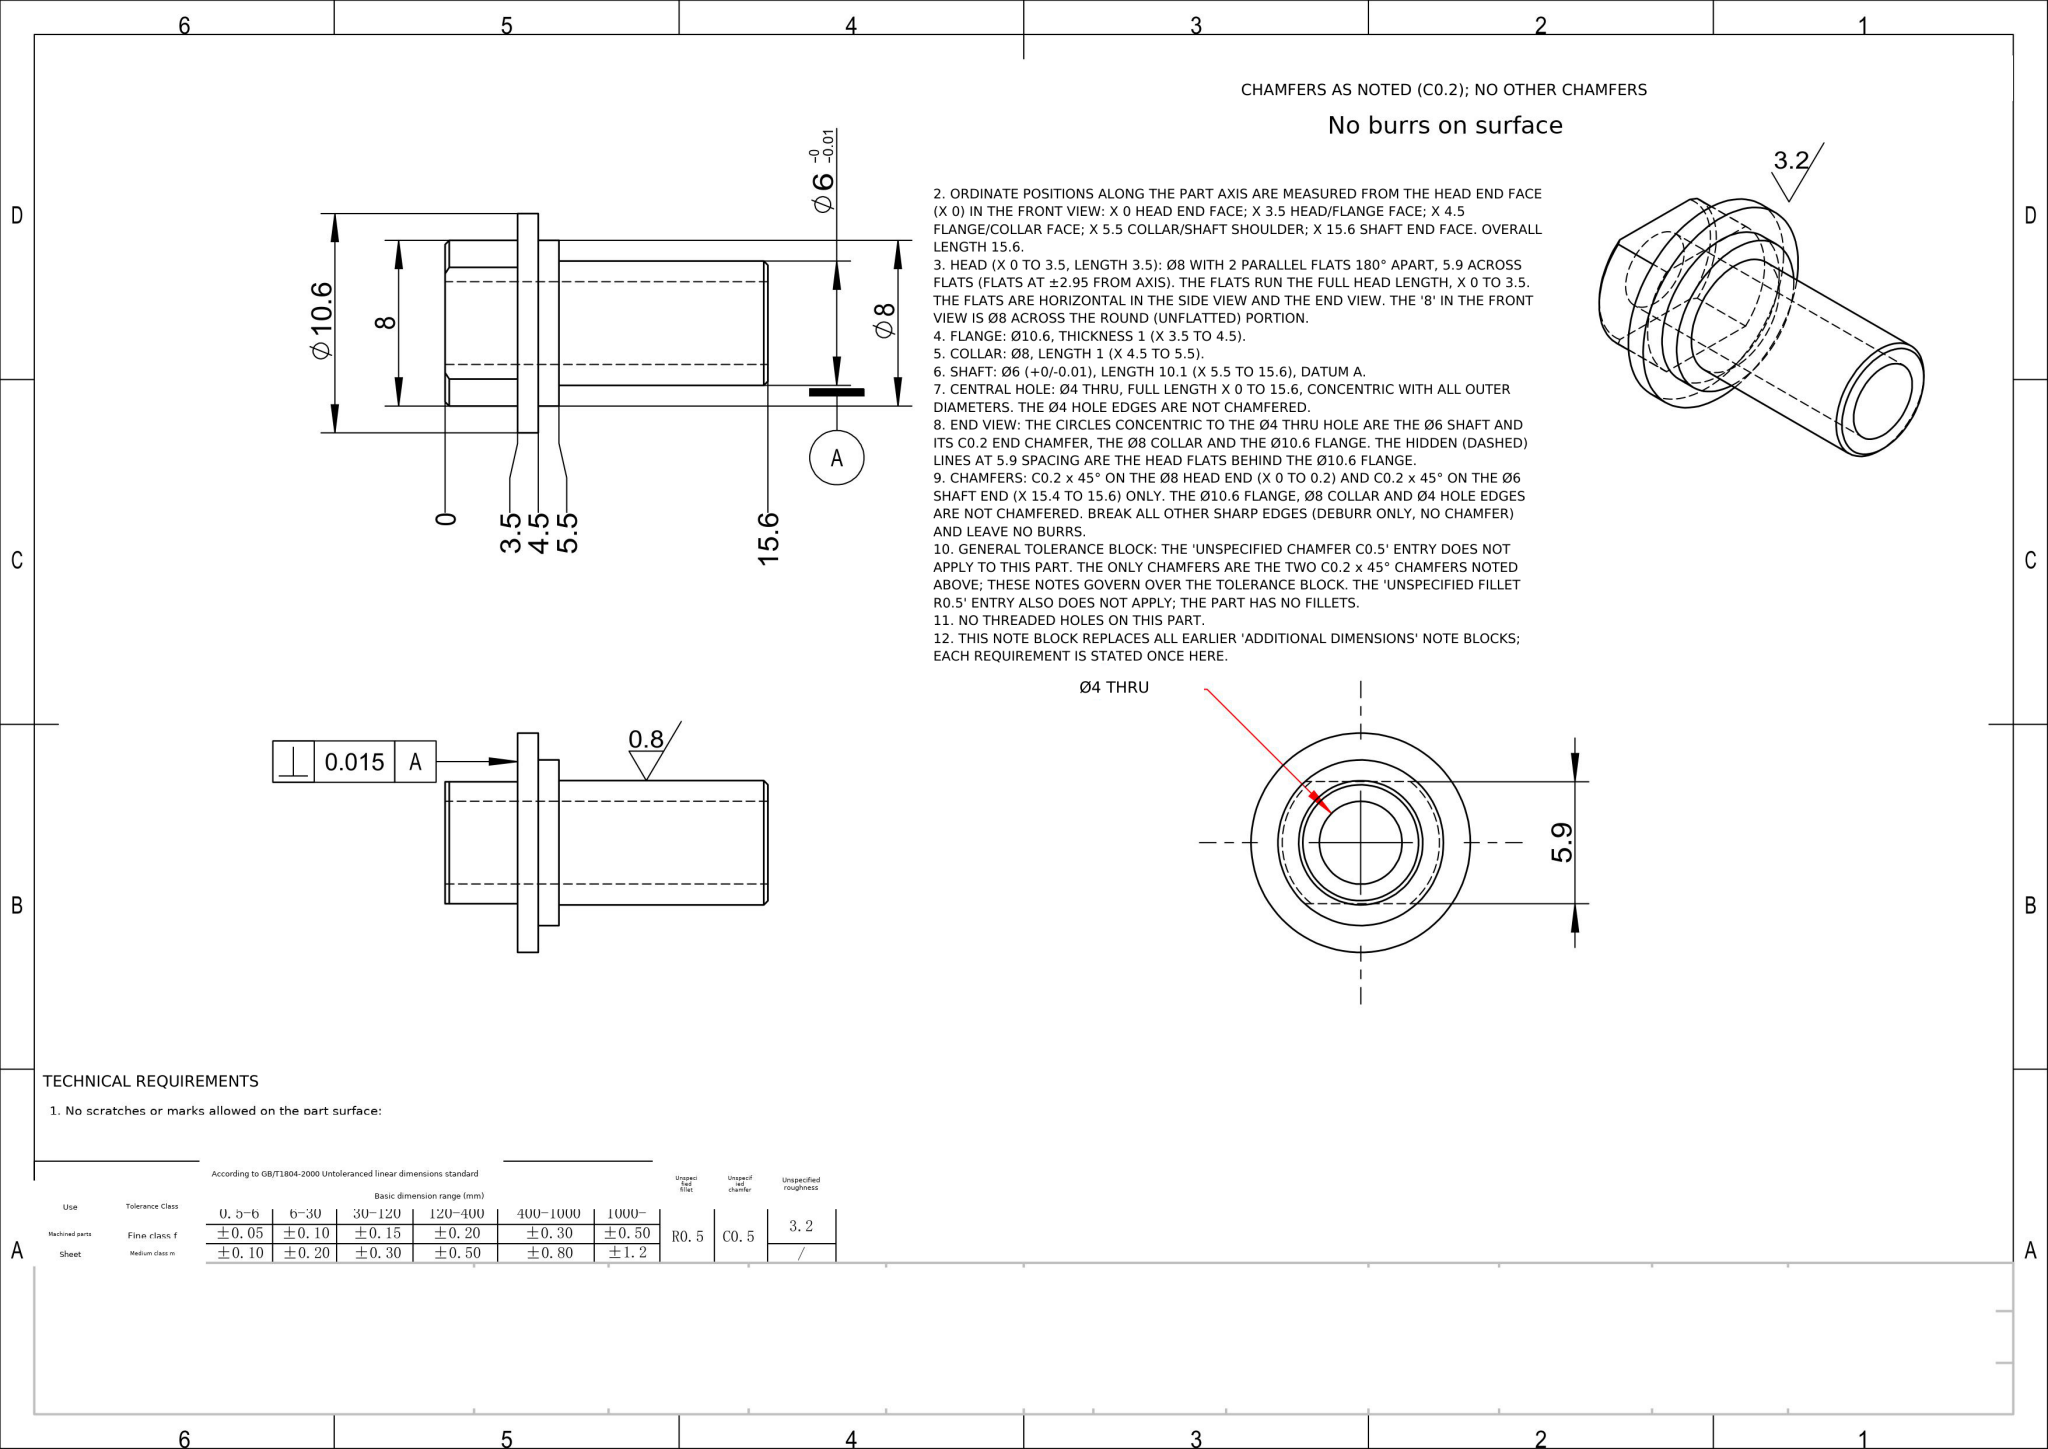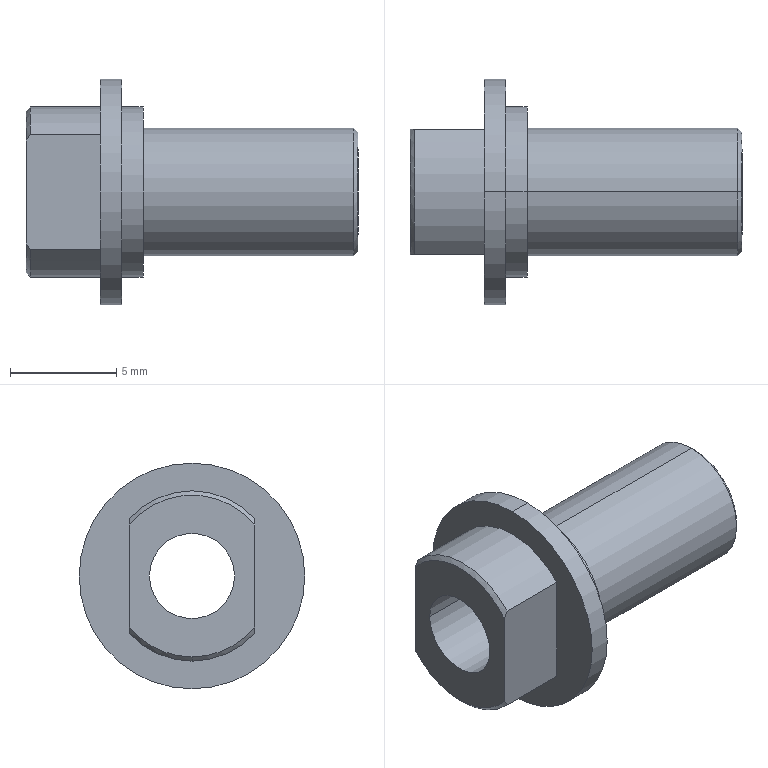Part | NX | mm | 1 solid | 23 faces | box 15.6 x 10.6 x 10.6 mm | volume 376 mm3 | cylinder 11 | plane 7 | cone 5 | commonest cylinder face diameters 8 x5 4 x2 6 x2 10.6 x2
STEP:
#1=COLOUR_RGB('',0.7529,0.7529,0.7529);
#2=FILL_AREA_STYLE_COLOUR('',#1);
#3=FILL_AREA_STYLE('',(#2));
#4=SURFACE_STYLE_FILL_AREA(#3);
#5=SURFACE_SIDE_STYLE('',(#4));
#6=SURFACE_STYLE_USAGE(.BOTH.,#5);
#7=PRESENTATION_STYLE_ASSIGNMENT((#6));
#8=CARTESIAN_POINT('',(-0.,-2.,0.));
#9=VERTEX_POINT('',#8);
#10=CARTESIAN_POINT('',(-0.,2.,0.));
#11=VERTEX_POINT('',#10);
#12=CARTESIAN_POINT('',(-0.,0.,0.));
#13=DIRECTION('',(1.,-0.,0.));
#14=DIRECTION('',(0.,1.,0.));
#15=AXIS2_PLACEMENT_3D('',#12,#13,#14);
#16=CIRCLE('',#15,2.);
#17=EDGE_CURVE('',#9,#11,#16,.T.);
#18=ORIENTED_EDGE('',*,*,#17,.F.);
#19=CARTESIAN_POINT('',(15.6,-2.,0.));
#20=VERTEX_POINT('',#19);
#21=CARTESIAN_POINT('',(-6.035,-2.,0.));
#22=DIRECTION('',(1.,-0.,0.));
#23=VECTOR('',#22,1000.);
#24=LINE('',#21,#23);
#25=EDGE_CURVE('',#9,#20,#24,.T.);
#26=ORIENTED_EDGE('',*,*,#25,.T.);
#27=CARTESIAN_POINT('',(15.6,2.,0.));
#28=VERTEX_POINT('',#27);
#29=CARTESIAN_POINT('',(15.6,-0.,0.));
#30=DIRECTION('',(-1.,0.,0.));
#31=DIRECTION('',(0.,1.,0.));
#32=AXIS2_PLACEMENT_3D('',#29,#30,#31);
#33=CIRCLE('',#32,2.);
#34=EDGE_CURVE('',#28,#20,#33,.T.);
#35=ORIENTED_EDGE('',*,*,#34,.F.);
#36=CARTESIAN_POINT('',(-6.035,2.,0.));
#37=DIRECTION('',(1.,-0.,0.));
#38=VECTOR('',#37,1000.);
#39=LINE('',#36,#38);
#40=EDGE_CURVE('',#11,#28,#39,.T.);
#41=ORIENTED_EDGE('',*,*,#40,.F.);
#42=EDGE_LOOP('',(#18,#26,#35,#41));
#43=FACE_OUTER_BOUND('',#42,.T.);
#44=CARTESIAN_POINT('',(-6.035,0.,0.));
#45=DIRECTION('',(1.,-0.,0.));
#46=DIRECTION('',(0.,1.,0.));
#47=AXIS2_PLACEMENT_3D('',#44,#45,#46);
#48=CYLINDRICAL_SURFACE('',#47,2.);
#49=ADVANCED_FACE('',(#43),#48,.F.);
#50=CARTESIAN_POINT('',(0.,0.,-3.8));
#51=VERTEX_POINT('',#50);
#52=CARTESIAN_POINT('',(-0.,-2.95,-2.395));
#53=VERTEX_POINT('',#52);
#54=CARTESIAN_POINT('',(0.,0.,0.));
#55=DIRECTION('',(-1.,0.,0.));
#56=DIRECTION('',(0.,0.,-1.));
#57=AXIS2_PLACEMENT_3D('',#54,#55,#56);
#58=CIRCLE('',#57,3.8);
#59=EDGE_CURVE('',#51,#53,#58,.T.);
#60=ORIENTED_EDGE('',*,*,#59,.F.);
#61=CARTESIAN_POINT('',(0.2,-0.,-4.));
#62=VERTEX_POINT('',#61);
#63=CARTESIAN_POINT('',(0.2,0.,-4.));
#64=DIRECTION('',(0.7071,0.,-0.7071));
#65=VECTOR('',#64,1000.);
#66=LINE('',#63,#65);
#67=EDGE_CURVE('',#51,#62,#66,.T.);
#68=ORIENTED_EDGE('',*,*,#67,.T.);
#69=CARTESIAN_POINT('',(0.2,-2.95,-2.701));
#70=VERTEX_POINT('',#69);
#71=CARTESIAN_POINT('',(0.2,-0.,0.));
#72=DIRECTION('',(-1.,0.,0.));
#73=DIRECTION('',(-0.,1.,0.));
#74=AXIS2_PLACEMENT_3D('',#71,#72,#73);
#75=CIRCLE('',#74,4.);
#76=EDGE_CURVE('',#62,#70,#75,.T.);
#77=ORIENTED_EDGE('',*,*,#76,.T.);
#78=CARTESIAN_POINT('',(0.2,-2.95,-2.701));
#79=CARTESIAN_POINT('',(0.1318,-2.95,-2.6));
#80=CARTESIAN_POINT('',(0.06499,-2.95,-2.498));
#81=CARTESIAN_POINT('',(-0.,-2.95,-2.395));
#82=B_SPLINE_CURVE_WITH_KNOTS('',3,(#78,#79,#80,#81),.UNSPECIFIED.,.F.,.F.,(4,4),(0.,0.0003656),.UNSPECIFIED.);
#83=EDGE_CURVE('',#70,#53,#82,.T.);
#84=ORIENTED_EDGE('',*,*,#83,.T.);
#85=EDGE_LOOP('',(#60,#68,#77,#84));
#86=FACE_OUTER_BOUND('',#85,.T.);
#87=CARTESIAN_POINT('',(0.2,0.,0.));
#88=DIRECTION('',(1.,0.,0.));
#89=DIRECTION('',(0.,0.,-1.));
#90=AXIS2_PLACEMENT_3D('',#87,#88,#89);
#91=CONICAL_SURFACE('',#90,4.,0.7854);
#92=ADVANCED_FACE('',(#86),#91,.T.);
#93=CARTESIAN_POINT('',(15.6,0.,-2.8));
#94=VERTEX_POINT('',#93);
#95=CARTESIAN_POINT('',(15.6,0.,2.8));
#96=VERTEX_POINT('',#95);
#97=CARTESIAN_POINT('',(15.6,0.,0.));
#98=DIRECTION('',(1.,0.,0.));
#99=DIRECTION('',(0.,0.,1.));
#100=AXIS2_PLACEMENT_3D('',#97,#98,#99);
#101=CIRCLE('',#100,2.8);
#102=EDGE_CURVE('',#94,#96,#101,.T.);
#103=ORIENTED_EDGE('',*,*,#102,.F.);
#104=CARTESIAN_POINT('',(15.4,-0.,-3.));
#105=VERTEX_POINT('',#104);
#106=CARTESIAN_POINT('',(15.4,0.,-3.));
#107=DIRECTION('',(-0.7071,0.,-0.7071));
#108=VECTOR('',#107,1000.);
#109=LINE('',#106,#108);
#110=EDGE_CURVE('',#94,#105,#109,.T.);
#111=ORIENTED_EDGE('',*,*,#110,.T.);
#112=CARTESIAN_POINT('',(15.4,0.,3.));
#113=VERTEX_POINT('',#112);
#114=CARTESIAN_POINT('',(15.4,-0.,0.));
#115=DIRECTION('',(1.,-0.,0.));
#116=DIRECTION('',(0.,-1.,0.));
#117=AXIS2_PLACEMENT_3D('',#114,#115,#116);
#118=CIRCLE('',#117,3.);
#119=EDGE_CURVE('',#105,#113,#118,.T.);
#120=ORIENTED_EDGE('',*,*,#119,.T.);
#121=CARTESIAN_POINT('',(15.4,0.,3.));
#122=DIRECTION('',(-0.7071,0.,0.7071));
#123=VECTOR('',#122,1000.);
#124=LINE('',#121,#123);
#125=EDGE_CURVE('',#96,#113,#124,.T.);
#126=ORIENTED_EDGE('',*,*,#125,.F.);
#127=EDGE_LOOP('',(#103,#111,#120,#126));
#128=FACE_OUTER_BOUND('',#127,.T.);
#129=CARTESIAN_POINT('',(15.4,0.,0.));
#130=DIRECTION('',(-1.,0.,0.));
#131=DIRECTION('',(0.,0.,1.));
#132=AXIS2_PLACEMENT_3D('',#129,#130,#131);
#133=CONICAL_SURFACE('',#132,3.,0.7854);
#134=ADVANCED_FACE('',(#128),#133,.T.);
#135=ORIENTED_EDGE('',*,*,#76,.F.);
#136=CARTESIAN_POINT('',(3.5,-0.,-4.));
#137=VERTEX_POINT('',#136);
#138=CARTESIAN_POINT('',(1.75,-0.,-4.));
#139=DIRECTION('',(1.,0.,0.));
#140=VECTOR('',#139,1000.);
#141=LINE('',#138,#140);
#142=EDGE_CURVE('',#62,#137,#141,.T.);
#143=ORIENTED_EDGE('',*,*,#142,.T.);
#144=CARTESIAN_POINT('',(3.5,-2.95,-2.701));
#145=VERTEX_POINT('',#144);
#146=CARTESIAN_POINT('',(3.5,-0.,0.));
#147=DIRECTION('',(-1.,0.,0.));
#148=DIRECTION('',(0.,0.,-1.));
#149=AXIS2_PLACEMENT_3D('',#146,#147,#148);
#150=CIRCLE('',#149,4.);
#151=EDGE_CURVE('',#137,#145,#150,.T.);
#152=ORIENTED_EDGE('',*,*,#151,.T.);
#153=CARTESIAN_POINT('',(-0.,-2.95,-2.701));
#154=DIRECTION('',(-1.,0.,0.));
#155=VECTOR('',#154,1000.);
#156=LINE('',#153,#155);
#157=EDGE_CURVE('',#145,#70,#156,.T.);
#158=ORIENTED_EDGE('',*,*,#157,.T.);
#159=EDGE_LOOP('',(#135,#143,#152,#158));
#160=FACE_OUTER_BOUND('',#159,.T.);
#161=CARTESIAN_POINT('',(1.75,-0.,0.));
#162=DIRECTION('',(1.,0.,0.));
#163=DIRECTION('',(0.,0.,-1.));
#164=AXIS2_PLACEMENT_3D('',#161,#162,#163);
#165=CYLINDRICAL_SURFACE('',#164,4.);
#166=ADVANCED_FACE('',(#160),#165,.T.);
#167=CARTESIAN_POINT('',(5.5,-0.,-3.));
#168=VERTEX_POINT('',#167);
#169=CARTESIAN_POINT('',(5.5,0.,3.));
#170=VERTEX_POINT('',#169);
#171=CARTESIAN_POINT('',(5.5,-0.,0.));
#172=DIRECTION('',(1.,0.,0.));
#173=DIRECTION('',(0.,0.,-1.));
#174=AXIS2_PLACEMENT_3D('',#171,#172,#173);
#175=CIRCLE('',#174,3.);
#176=EDGE_CURVE('',#168,#170,#175,.T.);
#177=ORIENTED_EDGE('',*,*,#176,.T.);
#178=CARTESIAN_POINT('',(10.55,0.,3.));
#179=DIRECTION('',(1.,0.,0.));
#180=VECTOR('',#179,1000.);
#181=LINE('',#178,#180);
#182=EDGE_CURVE('',#170,#113,#181,.T.);
#183=ORIENTED_EDGE('',*,*,#182,.T.);
#184=ORIENTED_EDGE('',*,*,#119,.F.);
#185=CARTESIAN_POINT('',(10.55,-0.,-3.));
#186=DIRECTION('',(1.,0.,0.));
#187=VECTOR('',#186,1000.);
#188=LINE('',#185,#187);
#189=EDGE_CURVE('',#168,#105,#188,.T.);
#190=ORIENTED_EDGE('',*,*,#189,.F.);
#191=EDGE_LOOP('',(#177,#183,#184,#190));
#192=FACE_OUTER_BOUND('',#191,.T.);
#193=CARTESIAN_POINT('',(10.55,-0.,0.));
#194=DIRECTION('',(1.,0.,0.));
#195=DIRECTION('',(0.,0.,-1.));
#196=AXIS2_PLACEMENT_3D('',#193,#194,#195);
#197=CYLINDRICAL_SURFACE('',#196,3.);
#198=ADVANCED_FACE('',(#192),#197,.T.);
#199=CARTESIAN_POINT('',(3.5,0.,5.3));
#200=VERTEX_POINT('',#199);
#201=CARTESIAN_POINT('',(3.5,-0.,-5.3));
#202=VERTEX_POINT('',#201);
#203=CARTESIAN_POINT('',(3.5,-0.,0.));
#204=DIRECTION('',(-1.,0.,0.));
#205=DIRECTION('',(0.,0.,-1.));
#206=AXIS2_PLACEMENT_3D('',#203,#204,#205);
#207=CIRCLE('',#206,5.3);
#208=EDGE_CURVE('',#200,#202,#207,.T.);
#209=ORIENTED_EDGE('',*,*,#208,.F.);
#210=CARTESIAN_POINT('',(4.5,0.,5.3));
#211=VERTEX_POINT('',#210);
#212=CARTESIAN_POINT('',(4.5,0.,5.3));
#213=DIRECTION('',(1.,0.,0.));
#214=VECTOR('',#213,1000.);
#215=LINE('',#212,#214);
#216=EDGE_CURVE('',#200,#211,#215,.T.);
#217=ORIENTED_EDGE('',*,*,#216,.T.);
#218=CARTESIAN_POINT('',(4.5,-0.,-5.3));
#219=VERTEX_POINT('',#218);
#220=CARTESIAN_POINT('',(4.5,-0.,0.));
#221=DIRECTION('',(-1.,0.,0.));
#222=DIRECTION('',(0.,0.,-1.));
#223=AXIS2_PLACEMENT_3D('',#220,#221,#222);
#224=CIRCLE('',#223,5.3);
#225=EDGE_CURVE('',#211,#219,#224,.T.);
#226=ORIENTED_EDGE('',*,*,#225,.T.);
#227=CARTESIAN_POINT('',(4.5,-0.,-5.3));
#228=DIRECTION('',(1.,0.,0.));
#229=VECTOR('',#228,1000.);
#230=LINE('',#227,#229);
#231=EDGE_CURVE('',#202,#219,#230,.T.);
#232=ORIENTED_EDGE('',*,*,#231,.F.);
#233=EDGE_LOOP('',(#209,#217,#226,#232));
#234=FACE_OUTER_BOUND('',#233,.T.);
#235=CARTESIAN_POINT('',(4.5,-0.,0.));
#236=DIRECTION('',(1.,0.,0.));
#237=DIRECTION('',(0.,0.,-1.));
#238=AXIS2_PLACEMENT_3D('',#235,#236,#237);
#239=CYLINDRICAL_SURFACE('',#238,5.3);
#240=ADVANCED_FACE('',(#234),#239,.T.);
#241=CARTESIAN_POINT('',(4.5,-0.,-4.));
#242=VERTEX_POINT('',#241);
#243=CARTESIAN_POINT('',(4.5,0.,4.));
#244=VERTEX_POINT('',#243);
#245=CARTESIAN_POINT('',(4.5,-0.,0.));
#246=DIRECTION('',(1.,0.,0.));
#247=DIRECTION('',(0.,0.,-1.));
#248=AXIS2_PLACEMENT_3D('',#245,#246,#247);
#249=CIRCLE('',#248,4.);
#250=EDGE_CURVE('',#242,#244,#249,.T.);
#251=ORIENTED_EDGE('',*,*,#250,.T.);
#252=CARTESIAN_POINT('',(5.5,0.,4.));
#253=VERTEX_POINT('',#252);
#254=CARTESIAN_POINT('',(5.,0.,4.));
#255=DIRECTION('',(1.,0.,0.));
#256=VECTOR('',#255,1000.);
#257=LINE('',#254,#256);
#258=EDGE_CURVE('',#244,#253,#257,.T.);
#259=ORIENTED_EDGE('',*,*,#258,.T.);
#260=CARTESIAN_POINT('',(5.5,-0.,-4.));
#261=VERTEX_POINT('',#260);
#262=CARTESIAN_POINT('',(5.5,-0.,0.));
#263=DIRECTION('',(1.,0.,0.));
#264=DIRECTION('',(0.,0.,-1.));
#265=AXIS2_PLACEMENT_3D('',#262,#263,#264);
#266=CIRCLE('',#265,4.);
#267=EDGE_CURVE('',#261,#253,#266,.T.);
#268=ORIENTED_EDGE('',*,*,#267,.F.);
#269=CARTESIAN_POINT('',(5.,-0.,-4.));
#270=DIRECTION('',(1.,0.,0.));
#271=VECTOR('',#270,1000.);
#272=LINE('',#269,#271);
#273=EDGE_CURVE('',#242,#261,#272,.T.);
#274=ORIENTED_EDGE('',*,*,#273,.F.);
#275=EDGE_LOOP('',(#251,#259,#268,#274));
#276=FACE_OUTER_BOUND('',#275,.T.);
#277=CARTESIAN_POINT('',(5.,-0.,0.));
#278=DIRECTION('',(1.,0.,0.));
#279=DIRECTION('',(0.,0.,-1.));
#280=AXIS2_PLACEMENT_3D('',#277,#278,#279);
#281=CYLINDRICAL_SURFACE('',#280,4.);
#282=ADVANCED_FACE('',(#276),#281,.T.);
#283=ORIENTED_EDGE('',*,*,#25,.F.);
#284=CARTESIAN_POINT('',(-0.,0.,0.));
#285=DIRECTION('',(1.,-0.,0.));
#286=DIRECTION('',(0.,1.,0.));
#287=AXIS2_PLACEMENT_3D('',#284,#285,#286);
#288=CIRCLE('',#287,2.);
#289=EDGE_CURVE('',#11,#9,#288,.T.);
#290=ORIENTED_EDGE('',*,*,#289,.F.);
#291=ORIENTED_EDGE('',*,*,#40,.T.);
#292=CARTESIAN_POINT('',(15.6,-0.,0.));
#293=DIRECTION('',(-1.,0.,0.));
#294=DIRECTION('',(0.,1.,0.));
#295=AXIS2_PLACEMENT_3D('',#292,#293,#294);
#296=CIRCLE('',#295,2.);
#297=EDGE_CURVE('',#20,#28,#296,.T.);
#298=ORIENTED_EDGE('',*,*,#297,.F.);
#299=EDGE_LOOP('',(#283,#290,#291,#298));
#300=FACE_OUTER_BOUND('',#299,.T.);
#301=CARTESIAN_POINT('',(-6.035,0.,0.));
#302=DIRECTION('',(1.,-0.,0.));
#303=DIRECTION('',(0.,1.,0.));
#304=AXIS2_PLACEMENT_3D('',#301,#302,#303);
#305=CYLINDRICAL_SURFACE('',#304,2.);
#306=ADVANCED_FACE('',(#300),#305,.F.);
#307=ORIENTED_EDGE('',*,*,#289,.T.);
#308=ORIENTED_EDGE('',*,*,#17,.T.);
#309=EDGE_LOOP('',(#307,#308));
#310=FACE_BOUND('',#309,.T.);
#311=CARTESIAN_POINT('',(-0.,2.95,-2.395));
#312=VERTEX_POINT('',#311);
#313=CARTESIAN_POINT('',(0.,0.,0.));
#314=DIRECTION('',(-1.,0.,0.));
#315=DIRECTION('',(0.,0.,-1.));
#316=AXIS2_PLACEMENT_3D('',#313,#314,#315);
#317=CIRCLE('',#316,3.8);
#318=EDGE_CURVE('',#312,#51,#317,.T.);
#319=ORIENTED_EDGE('',*,*,#318,.T.);
#320=ORIENTED_EDGE('',*,*,#59,.T.);
#321=CARTESIAN_POINT('',(-0.,-2.95,2.395));
#322=VERTEX_POINT('',#321);
#323=CARTESIAN_POINT('',(-0.,-2.95,0.));
#324=DIRECTION('',(0.,0.,1.));
#325=VECTOR('',#324,1000.);
#326=LINE('',#323,#325);
#327=EDGE_CURVE('',#53,#322,#326,.T.);
#328=ORIENTED_EDGE('',*,*,#327,.T.);
#329=CARTESIAN_POINT('',(-0.,2.95,2.395));
#330=VERTEX_POINT('',#329);
#331=CARTESIAN_POINT('',(0.,0.,0.));
#332=DIRECTION('',(-1.,0.,0.));
#333=DIRECTION('',(0.,0.,-1.));
#334=AXIS2_PLACEMENT_3D('',#331,#332,#333);
#335=CIRCLE('',#334,3.8);
#336=EDGE_CURVE('',#322,#330,#335,.T.);
#337=ORIENTED_EDGE('',*,*,#336,.T.);
#338=CARTESIAN_POINT('',(-0.,2.95,0.));
#339=DIRECTION('',(0.,0.,-1.));
#340=VECTOR('',#339,1000.);
#341=LINE('',#338,#340);
#342=EDGE_CURVE('',#330,#312,#341,.T.);
#343=ORIENTED_EDGE('',*,*,#342,.T.);
#344=EDGE_LOOP('',(#319,#320,#328,#337,#343));
#345=FACE_OUTER_BOUND('',#344,.T.);
#346=CARTESIAN_POINT('',(-0.,2.,0.));
#347=DIRECTION('',(-1.,0.,0.));
#348=DIRECTION('',(-0.,-1.,0.));
#349=AXIS2_PLACEMENT_3D('',#346,#347,#348);
#350=PLANE('',#349);
#351=ADVANCED_FACE('',(#310,#345),#350,.T.);
#352=ORIENTED_EDGE('',*,*,#34,.T.);
#353=ORIENTED_EDGE('',*,*,#297,.T.);
#354=EDGE_LOOP('',(#352,#353));
#355=FACE_BOUND('',#354,.T.);
#356=CARTESIAN_POINT('',(15.6,0.,0.));
#357=DIRECTION('',(1.,0.,0.));
#358=DIRECTION('',(0.,0.,1.));
#359=AXIS2_PLACEMENT_3D('',#356,#357,#358);
#360=CIRCLE('',#359,2.8);
#361=EDGE_CURVE('',#96,#94,#360,.T.);
#362=ORIENTED_EDGE('',*,*,#361,.T.);
#363=ORIENTED_EDGE('',*,*,#102,.T.);
#364=EDGE_LOOP('',(#362,#363));
#365=FACE_OUTER_BOUND('',#364,.T.);
#366=CARTESIAN_POINT('',(15.6,1.5,0.));
#367=DIRECTION('',(1.,-0.,0.));
#368=DIRECTION('',(0.,1.,0.));
#369=AXIS2_PLACEMENT_3D('',#366,#367,#368);
#370=PLANE('',#369);
#371=ADVANCED_FACE('',(#355,#365),#370,.T.);
#372=ORIENTED_EDGE('',*,*,#327,.F.);
#373=ORIENTED_EDGE('',*,*,#83,.F.);
#374=ORIENTED_EDGE('',*,*,#157,.F.);
#375=CARTESIAN_POINT('',(3.5,-2.95,2.701));
#376=VERTEX_POINT('',#375);
#377=CARTESIAN_POINT('',(3.5,-2.95,2.701));
#378=DIRECTION('',(0.,0.,-1.));
#379=VECTOR('',#378,1000.);
#380=LINE('',#377,#379);
#381=EDGE_CURVE('',#376,#145,#380,.T.);
#382=ORIENTED_EDGE('',*,*,#381,.F.);
#383=CARTESIAN_POINT('',(0.2,-2.95,2.701));
#384=VERTEX_POINT('',#383);
#385=CARTESIAN_POINT('',(-0.,-2.95,2.701));
#386=DIRECTION('',(1.,0.,0.));
#387=VECTOR('',#386,1000.);
#388=LINE('',#385,#387);
#389=EDGE_CURVE('',#384,#376,#388,.T.);
#390=ORIENTED_EDGE('',*,*,#389,.F.);
#391=CARTESIAN_POINT('',(-0.,-2.95,2.395));
#392=CARTESIAN_POINT('',(0.06499,-2.95,2.498));
#393=CARTESIAN_POINT('',(0.1318,-2.95,2.6));
#394=CARTESIAN_POINT('',(0.2,-2.95,2.701));
#395=B_SPLINE_CURVE_WITH_KNOTS('',3,(#391,#392,#393,#394),.UNSPECIFIED.,.F.,.F.,(4,4),(0.,0.0003656),.UNSPECIFIED.);
#396=EDGE_CURVE('',#322,#384,#395,.T.);
#397=ORIENTED_EDGE('',*,*,#396,.F.);
#398=EDGE_LOOP('',(#372,#373,#374,#382,#390,#397));
#399=FACE_OUTER_BOUND('',#398,.T.);
#400=CARTESIAN_POINT('',(-0.,-2.95,2.701));
#401=DIRECTION('',(0.,1.,0.));
#402=DIRECTION('',(0.,0.,1.));
#403=AXIS2_PLACEMENT_3D('',#400,#401,#402);
#404=PLANE('',#403);
#405=ADVANCED_FACE('',(#399),#404,.F.);
#406=ORIENTED_EDGE('',*,*,#67,.F.);
#407=ORIENTED_EDGE('',*,*,#318,.F.);
#408=CARTESIAN_POINT('',(0.2,2.95,-2.701));
#409=VERTEX_POINT('',#408);
#410=CARTESIAN_POINT('',(-0.,2.95,-2.395));
#411=CARTESIAN_POINT('',(0.06499,2.95,-2.498));
#412=CARTESIAN_POINT('',(0.1318,2.95,-2.6));
#413=CARTESIAN_POINT('',(0.2,2.95,-2.701));
#414=B_SPLINE_CURVE_WITH_KNOTS('',3,(#410,#411,#412,#413),.UNSPECIFIED.,.F.,.F.,(4,4),(0.,0.0003656),.UNSPECIFIED.);
#415=EDGE_CURVE('',#312,#409,#414,.T.);
#416=ORIENTED_EDGE('',*,*,#415,.T.);
#417=CARTESIAN_POINT('',(0.2,-0.,0.));
#418=DIRECTION('',(-1.,0.,0.));
#419=DIRECTION('',(-0.,1.,0.));
#420=AXIS2_PLACEMENT_3D('',#417,#418,#419);
#421=CIRCLE('',#420,4.);
#422=EDGE_CURVE('',#409,#62,#421,.T.);
#423=ORIENTED_EDGE('',*,*,#422,.T.);
#424=EDGE_LOOP('',(#406,#407,#416,#423));
#425=FACE_OUTER_BOUND('',#424,.T.);
#426=CARTESIAN_POINT('',(0.2,0.,0.));
#427=DIRECTION('',(1.,0.,0.));
#428=DIRECTION('',(0.,0.,-1.));
#429=AXIS2_PLACEMENT_3D('',#426,#427,#428);
#430=CONICAL_SURFACE('',#429,4.,0.7854);
#431=ADVANCED_FACE('',(#425),#430,.T.);
#432=CARTESIAN_POINT('',(3.5,2.95,2.701));
#433=VERTEX_POINT('',#432);
#434=CARTESIAN_POINT('',(0.2,2.95,2.701));
#435=VERTEX_POINT('',#434);
#436=CARTESIAN_POINT('',(-0.,2.95,2.701));
#437=DIRECTION('',(-1.,0.,0.));
#438=VECTOR('',#437,1000.);
#439=LINE('',#436,#438);
#440=EDGE_CURVE('',#433,#435,#439,.T.);
#441=ORIENTED_EDGE('',*,*,#440,.F.);
#442=CARTESIAN_POINT('',(3.5,2.95,-2.701));
#443=VERTEX_POINT('',#442);
#444=CARTESIAN_POINT('',(3.5,2.95,-2.701));
#445=DIRECTION('',(0.,0.,1.));
#446=VECTOR('',#445,1000.);
#447=LINE('',#444,#446);
#448=EDGE_CURVE('',#443,#433,#447,.T.);
#449=ORIENTED_EDGE('',*,*,#448,.F.);
#450=CARTESIAN_POINT('',(-0.,2.95,-2.701));
#451=DIRECTION('',(1.,0.,0.));
#452=VECTOR('',#451,1000.);
#453=LINE('',#450,#452);
#454=EDGE_CURVE('',#409,#443,#453,.T.);
#455=ORIENTED_EDGE('',*,*,#454,.F.);
#456=ORIENTED_EDGE('',*,*,#415,.F.);
#457=ORIENTED_EDGE('',*,*,#342,.F.);
#458=CARTESIAN_POINT('',(0.2,2.95,2.701));
#459=CARTESIAN_POINT('',(0.1318,2.95,2.6));
#460=CARTESIAN_POINT('',(0.06499,2.95,2.498));
#461=CARTESIAN_POINT('',(-0.,2.95,2.395));
#462=B_SPLINE_CURVE_WITH_KNOTS('',3,(#458,#459,#460,#461),.UNSPECIFIED.,.F.,.F.,(4,4),(0.,0.0003656),.UNSPECIFIED.);
#463=EDGE_CURVE('',#435,#330,#462,.T.);
#464=ORIENTED_EDGE('',*,*,#463,.F.);
#465=EDGE_LOOP('',(#441,#449,#455,#456,#457,#464));
#466=FACE_OUTER_BOUND('',#465,.T.);
#467=CARTESIAN_POINT('',(-0.,2.95,-2.701));
#468=DIRECTION('',(0.,-1.,0.));
#469=DIRECTION('',(0.,0.,-1.));
#470=AXIS2_PLACEMENT_3D('',#467,#468,#469);
#471=PLANE('',#470);
#472=ADVANCED_FACE('',(#466),#471,.F.);
#473=ORIENTED_EDGE('',*,*,#463,.T.);
#474=ORIENTED_EDGE('',*,*,#336,.F.);
#475=ORIENTED_EDGE('',*,*,#396,.T.);
#476=CARTESIAN_POINT('',(0.2,-0.,0.));
#477=DIRECTION('',(-1.,0.,0.));
#478=DIRECTION('',(-0.,1.,0.));
#479=AXIS2_PLACEMENT_3D('',#476,#477,#478);
#480=CIRCLE('',#479,4.);
#481=EDGE_CURVE('',#384,#435,#480,.T.);
#482=ORIENTED_EDGE('',*,*,#481,.T.);
#483=EDGE_LOOP('',(#473,#474,#475,#482));
#484=FACE_OUTER_BOUND('',#483,.T.);
#485=CARTESIAN_POINT('',(0.2,0.,0.));
#486=DIRECTION('',(1.,0.,0.));
#487=DIRECTION('',(0.,0.,-1.));
#488=AXIS2_PLACEMENT_3D('',#485,#486,#487);
#489=CONICAL_SURFACE('',#488,4.,0.7854);
#490=ADVANCED_FACE('',(#484),#489,.T.);
#491=ORIENTED_EDGE('',*,*,#110,.F.);
#492=ORIENTED_EDGE('',*,*,#361,.F.);
#493=ORIENTED_EDGE('',*,*,#125,.T.);
#494=CARTESIAN_POINT('',(15.4,-0.,0.));
#495=DIRECTION('',(1.,-0.,0.));
#496=DIRECTION('',(0.,-1.,0.));
#497=AXIS2_PLACEMENT_3D('',#494,#495,#496);
#498=CIRCLE('',#497,3.);
#499=EDGE_CURVE('',#113,#105,#498,.T.);
#500=ORIENTED_EDGE('',*,*,#499,.T.);
#501=EDGE_LOOP('',(#491,#492,#493,#500));
#502=FACE_OUTER_BOUND('',#501,.T.);
#503=CARTESIAN_POINT('',(15.4,0.,0.));
#504=DIRECTION('',(-1.,0.,0.));
#505=DIRECTION('',(0.,0.,1.));
#506=AXIS2_PLACEMENT_3D('',#503,#504,#505);
#507=CONICAL_SURFACE('',#506,3.,0.7854);
#508=ADVANCED_FACE('',(#502),#507,.T.);
#509=ORIENTED_EDGE('',*,*,#142,.F.);
#510=ORIENTED_EDGE('',*,*,#422,.F.);
#511=ORIENTED_EDGE('',*,*,#454,.T.);
#512=CARTESIAN_POINT('',(3.5,-0.,0.));
#513=DIRECTION('',(-1.,0.,0.));
#514=DIRECTION('',(0.,-0.,-1.));
#515=AXIS2_PLACEMENT_3D('',#512,#513,#514);
#516=CIRCLE('',#515,4.);
#517=EDGE_CURVE('',#443,#137,#516,.T.);
#518=ORIENTED_EDGE('',*,*,#517,.T.);
#519=EDGE_LOOP('',(#509,#510,#511,#518));
#520=FACE_OUTER_BOUND('',#519,.T.);
#521=CARTESIAN_POINT('',(1.75,-0.,0.));
#522=DIRECTION('',(1.,0.,0.));
#523=DIRECTION('',(0.,0.,-1.));
#524=AXIS2_PLACEMENT_3D('',#521,#522,#523);
#525=CYLINDRICAL_SURFACE('',#524,4.);
#526=ADVANCED_FACE('',(#520),#525,.T.);
#527=ORIENTED_EDGE('',*,*,#517,.F.);
#528=ORIENTED_EDGE('',*,*,#448,.T.);
#529=CARTESIAN_POINT('',(3.5,-0.,0.));
#530=DIRECTION('',(1.,0.,0.));
#531=DIRECTION('',(0.,0.,-1.));
#532=AXIS2_PLACEMENT_3D('',#529,#530,#531);
#533=CIRCLE('',#532,4.);
#534=EDGE_CURVE('',#433,#376,#533,.T.);
#535=ORIENTED_EDGE('',*,*,#534,.T.);
#536=ORIENTED_EDGE('',*,*,#381,.T.);
#537=ORIENTED_EDGE('',*,*,#151,.F.);
#538=EDGE_LOOP('',(#527,#528,#535,#536,#537));
#539=FACE_BOUND('',#538,.T.);
#540=CARTESIAN_POINT('',(3.5,-0.,0.));
#541=DIRECTION('',(-1.,0.,0.));
#542=DIRECTION('',(0.,0.,-1.));
#543=AXIS2_PLACEMENT_3D('',#540,#541,#542);
#544=CIRCLE('',#543,5.3);
#545=EDGE_CURVE('',#202,#200,#544,.T.);
#546=ORIENTED_EDGE('',*,*,#545,.T.);
#547=ORIENTED_EDGE('',*,*,#208,.T.);
#548=EDGE_LOOP('',(#546,#547));
#549=FACE_OUTER_BOUND('',#548,.T.);
#550=CARTESIAN_POINT('',(3.5,2.65,0.));
#551=DIRECTION('',(-1.,0.,0.));
#552=DIRECTION('',(-0.,-1.,0.));
#553=AXIS2_PLACEMENT_3D('',#550,#551,#552);
#554=PLANE('',#553);
#555=ADVANCED_FACE('',(#539,#549),#554,.T.);
#556=ORIENTED_EDGE('',*,*,#534,.F.);
#557=ORIENTED_EDGE('',*,*,#440,.T.);
#558=ORIENTED_EDGE('',*,*,#481,.F.);
#559=ORIENTED_EDGE('',*,*,#389,.T.);
#560=EDGE_LOOP('',(#556,#557,#558,#559));
#561=FACE_OUTER_BOUND('',#560,.T.);
#562=CARTESIAN_POINT('',(1.75,-0.,0.));
#563=DIRECTION('',(1.,0.,0.));
#564=DIRECTION('',(0.,0.,-1.));
#565=AXIS2_PLACEMENT_3D('',#562,#563,#564);
#566=CYLINDRICAL_SURFACE('',#565,4.);
#567=ADVANCED_FACE('',(#561),#566,.T.);
#568=ORIENTED_EDGE('',*,*,#182,.F.);
#569=CARTESIAN_POINT('',(5.5,-0.,0.));
#570=DIRECTION('',(1.,0.,0.));
#571=DIRECTION('',(0.,0.,-1.));
#572=AXIS2_PLACEMENT_3D('',#569,#570,#571);
#573=CIRCLE('',#572,3.);
#574=EDGE_CURVE('',#170,#168,#573,.T.);
#575=ORIENTED_EDGE('',*,*,#574,.T.);
#576=ORIENTED_EDGE('',*,*,#189,.T.);
#577=ORIENTED_EDGE('',*,*,#499,.F.);
#578=EDGE_LOOP('',(#568,#575,#576,#577));
#579=FACE_OUTER_BOUND('',#578,.T.);
#580=CARTESIAN_POINT('',(10.55,-0.,0.));
#581=DIRECTION('',(1.,0.,0.));
#582=DIRECTION('',(0.,0.,-1.));
#583=AXIS2_PLACEMENT_3D('',#580,#581,#582);
#584=CYLINDRICAL_SURFACE('',#583,3.);
#585=ADVANCED_FACE('',(#579),#584,.T.);
#586=ORIENTED_EDGE('',*,*,#216,.F.);
#587=ORIENTED_EDGE('',*,*,#545,.F.);
#588=ORIENTED_EDGE('',*,*,#231,.T.);
#589=CARTESIAN_POINT('',(4.5,-0.,0.));
#590=DIRECTION('',(-1.,0.,0.));
#591=DIRECTION('',(0.,0.,-1.));
#592=AXIS2_PLACEMENT_3D('',#589,#590,#591);
#593=CIRCLE('',#592,5.3);
#594=EDGE_CURVE('',#219,#211,#593,.T.);
#595=ORIENTED_EDGE('',*,*,#594,.T.);
#596=EDGE_LOOP('',(#586,#587,#588,#595));
#597=FACE_OUTER_BOUND('',#596,.T.);
#598=CARTESIAN_POINT('',(4.5,-0.,0.));
#599=DIRECTION('',(1.,0.,0.));
#600=DIRECTION('',(0.,0.,-1.));
#601=AXIS2_PLACEMENT_3D('',#598,#599,#600);
#602=CYLINDRICAL_SURFACE('',#601,5.3);
#603=ADVANCED_FACE('',(#597),#602,.T.);
#604=ORIENTED_EDGE('',*,*,#176,.F.);
#605=ORIENTED_EDGE('',*,*,#574,.F.);
#606=EDGE_LOOP('',(#604,#605));
#607=FACE_BOUND('',#606,.T.);
#608=ORIENTED_EDGE('',*,*,#267,.T.);
#609=CARTESIAN_POINT('',(5.5,-0.,0.));
#610=DIRECTION('',(1.,0.,0.));
#611=DIRECTION('',(0.,0.,-1.));
#612=AXIS2_PLACEMENT_3D('',#609,#610,#611);
#613=CIRCLE('',#612,4.);
#614=EDGE_CURVE('',#253,#261,#613,.T.);
#615=ORIENTED_EDGE('',*,*,#614,.T.);
#616=EDGE_LOOP('',(#608,#615));
#617=FACE_OUTER_BOUND('',#616,.T.);
#618=CARTESIAN_POINT('',(5.5,2.65,0.));
#619=DIRECTION('',(1.,-0.,0.));
#620=DIRECTION('',(0.,1.,0.));
#621=AXIS2_PLACEMENT_3D('',#618,#619,#620);
#622=PLANE('',#621);
#623=ADVANCED_FACE('',(#607,#617),#622,.T.);
#624=ORIENTED_EDGE('',*,*,#250,.F.);
#625=CARTESIAN_POINT('',(4.5,-0.,0.));
#626=DIRECTION('',(1.,0.,0.));
#627=DIRECTION('',(0.,0.,-1.));
#628=AXIS2_PLACEMENT_3D('',#625,#626,#627);
#629=CIRCLE('',#628,4.);
#630=EDGE_CURVE('',#244,#242,#629,.T.);
#631=ORIENTED_EDGE('',*,*,#630,.F.);
#632=EDGE_LOOP('',(#624,#631));
#633=FACE_BOUND('',#632,.T.);
#634=ORIENTED_EDGE('',*,*,#594,.F.);
#635=ORIENTED_EDGE('',*,*,#225,.F.);
#636=EDGE_LOOP('',(#634,#635));
#637=FACE_OUTER_BOUND('',#636,.T.);
#638=CARTESIAN_POINT('',(4.5,4.65,0.));
#639=DIRECTION('',(-1.,0.,0.));
#640=DIRECTION('',(-0.,-1.,0.));
#641=AXIS2_PLACEMENT_3D('',#638,#639,#640);
#642=PLANE('',#641);
#643=ADVANCED_FACE('',(#633,#637),#642,.F.);
#644=ORIENTED_EDGE('',*,*,#258,.F.);
#645=ORIENTED_EDGE('',*,*,#630,.T.);
#646=ORIENTED_EDGE('',*,*,#273,.T.);
#647=ORIENTED_EDGE('',*,*,#614,.F.);
#648=EDGE_LOOP('',(#644,#645,#646,#647));
#649=FACE_OUTER_BOUND('',#648,.T.);
#650=CARTESIAN_POINT('',(5.,-0.,0.));
#651=DIRECTION('',(1.,0.,0.));
#652=DIRECTION('',(0.,0.,-1.));
#653=AXIS2_PLACEMENT_3D('',#650,#651,#652);
#654=CYLINDRICAL_SURFACE('',#653,4.);
#655=ADVANCED_FACE('',(#649),#654,.T.);
#656=CLOSED_SHELL('',(#49,#92,#134,#166,#198,#240,#282,#306,#351,#371,#405,#431,#472,#490,#508,#526,#555,#567,#585,#603,#623,#643,#655));
#657=MANIFOLD_SOLID_BREP('',#656);
#658=STYLED_ITEM('',(#7),#657);
#659=(LENGTH_UNIT()NAMED_UNIT(*)SI_UNIT(.MILLI.,.METRE.));
#660=UNCERTAINTY_MEASURE_WITH_UNIT(LENGTH_MEASURE(0.00001),#659,'','');
#661=(NAMED_UNIT(*)PLANE_ANGLE_UNIT()SI_UNIT($,.RADIAN.));
#662=(NAMED_UNIT(*)SI_UNIT($,.STERADIAN.)SOLID_ANGLE_UNIT());
#663=(GEOMETRIC_REPRESENTATION_CONTEXT(3)GLOBAL_UNCERTAINTY_ASSIGNED_CONTEXT((#660))GLOBAL_UNIT_ASSIGNED_CONTEXT((#659,#661,#662))REPRESENTATION_CONTEXT('',''));
#664=MECHANICAL_DESIGN_GEOMETRIC_PRESENTATION_REPRESENTATION('',(#658),#663);
#665=PRESENTATION_LAYER_ASSIGNMENT('','',(#658));
#666=COLOUR_RGB('',0.7529,0.7529,0.7529);
#667=FILL_AREA_STYLE_COLOUR('',#666);
#668=FILL_AREA_STYLE('',(#667));
#669=SURFACE_STYLE_FILL_AREA(#668);
#670=SURFACE_SIDE_STYLE('',(#669));
#671=SURFACE_STYLE_USAGE(.BOTH.,#670);
#672=PRESENTATION_STYLE_ASSIGNMENT((#671));
#673=CARTESIAN_POINT('',(0.,0.,0.));
#674=DIRECTION('',(0.,0.,1.));
#675=DIRECTION('',(1.,0.,0.));
#676=AXIS2_PLACEMENT_3D('',#673,#674,#675);
#677=(LENGTH_UNIT()NAMED_UNIT(*)SI_UNIT(.MILLI.,.METRE.));
#678=UNCERTAINTY_MEASURE_WITH_UNIT(LENGTH_MEASURE(0.00001),#677,'','');
#679=(NAMED_UNIT(*)PLANE_ANGLE_UNIT()SI_UNIT($,.RADIAN.));
#680=(NAMED_UNIT(*)SI_UNIT($,.STERADIAN.)SOLID_ANGLE_UNIT());
#681=(GEOMETRIC_REPRESENTATION_CONTEXT(3)GLOBAL_UNCERTAINTY_ASSIGNED_CONTEXT((#678))GLOBAL_UNIT_ASSIGNED_CONTEXT((#677,#679,#680))REPRESENTATION_CONTEXT('',''));
#682=ADVANCED_BREP_SHAPE_REPRESENTATION('',(#657,#676),#681);
#683=STYLED_ITEM('',(#672),#682);
#684=(LENGTH_UNIT()NAMED_UNIT(*)SI_UNIT(.MILLI.,.METRE.));
#685=UNCERTAINTY_MEASURE_WITH_UNIT(LENGTH_MEASURE(0.00001),#684,'','');
#686=(NAMED_UNIT(*)PLANE_ANGLE_UNIT()SI_UNIT($,.RADIAN.));
#687=(NAMED_UNIT(*)SI_UNIT($,.STERADIAN.)SOLID_ANGLE_UNIT());
#688=(GEOMETRIC_REPRESENTATION_CONTEXT(3)GLOBAL_UNCERTAINTY_ASSIGNED_CONTEXT((#685))GLOBAL_UNIT_ASSIGNED_CONTEXT((#684,#686,#687))REPRESENTATION_CONTEXT('',''));
#689=MECHANICAL_DESIGN_GEOMETRIC_PRESENTATION_REPRESENTATION('',(#683),#688);
#690=PRESENTATION_LAYER_ASSIGNMENT('','',(#683));